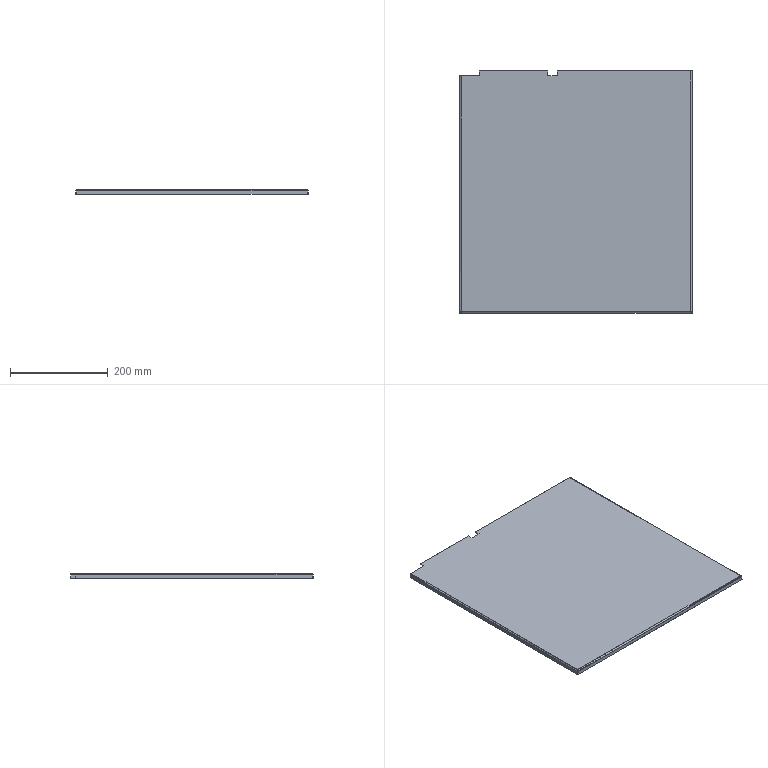Component | SolidWorks | PartitionRight-1 | 1 solid | 36 faces | volume 296314 mm3 | plane 26 | cylinder 6 | spline 4 | commonest cylinder face diameters 5.4 x3 3 x3